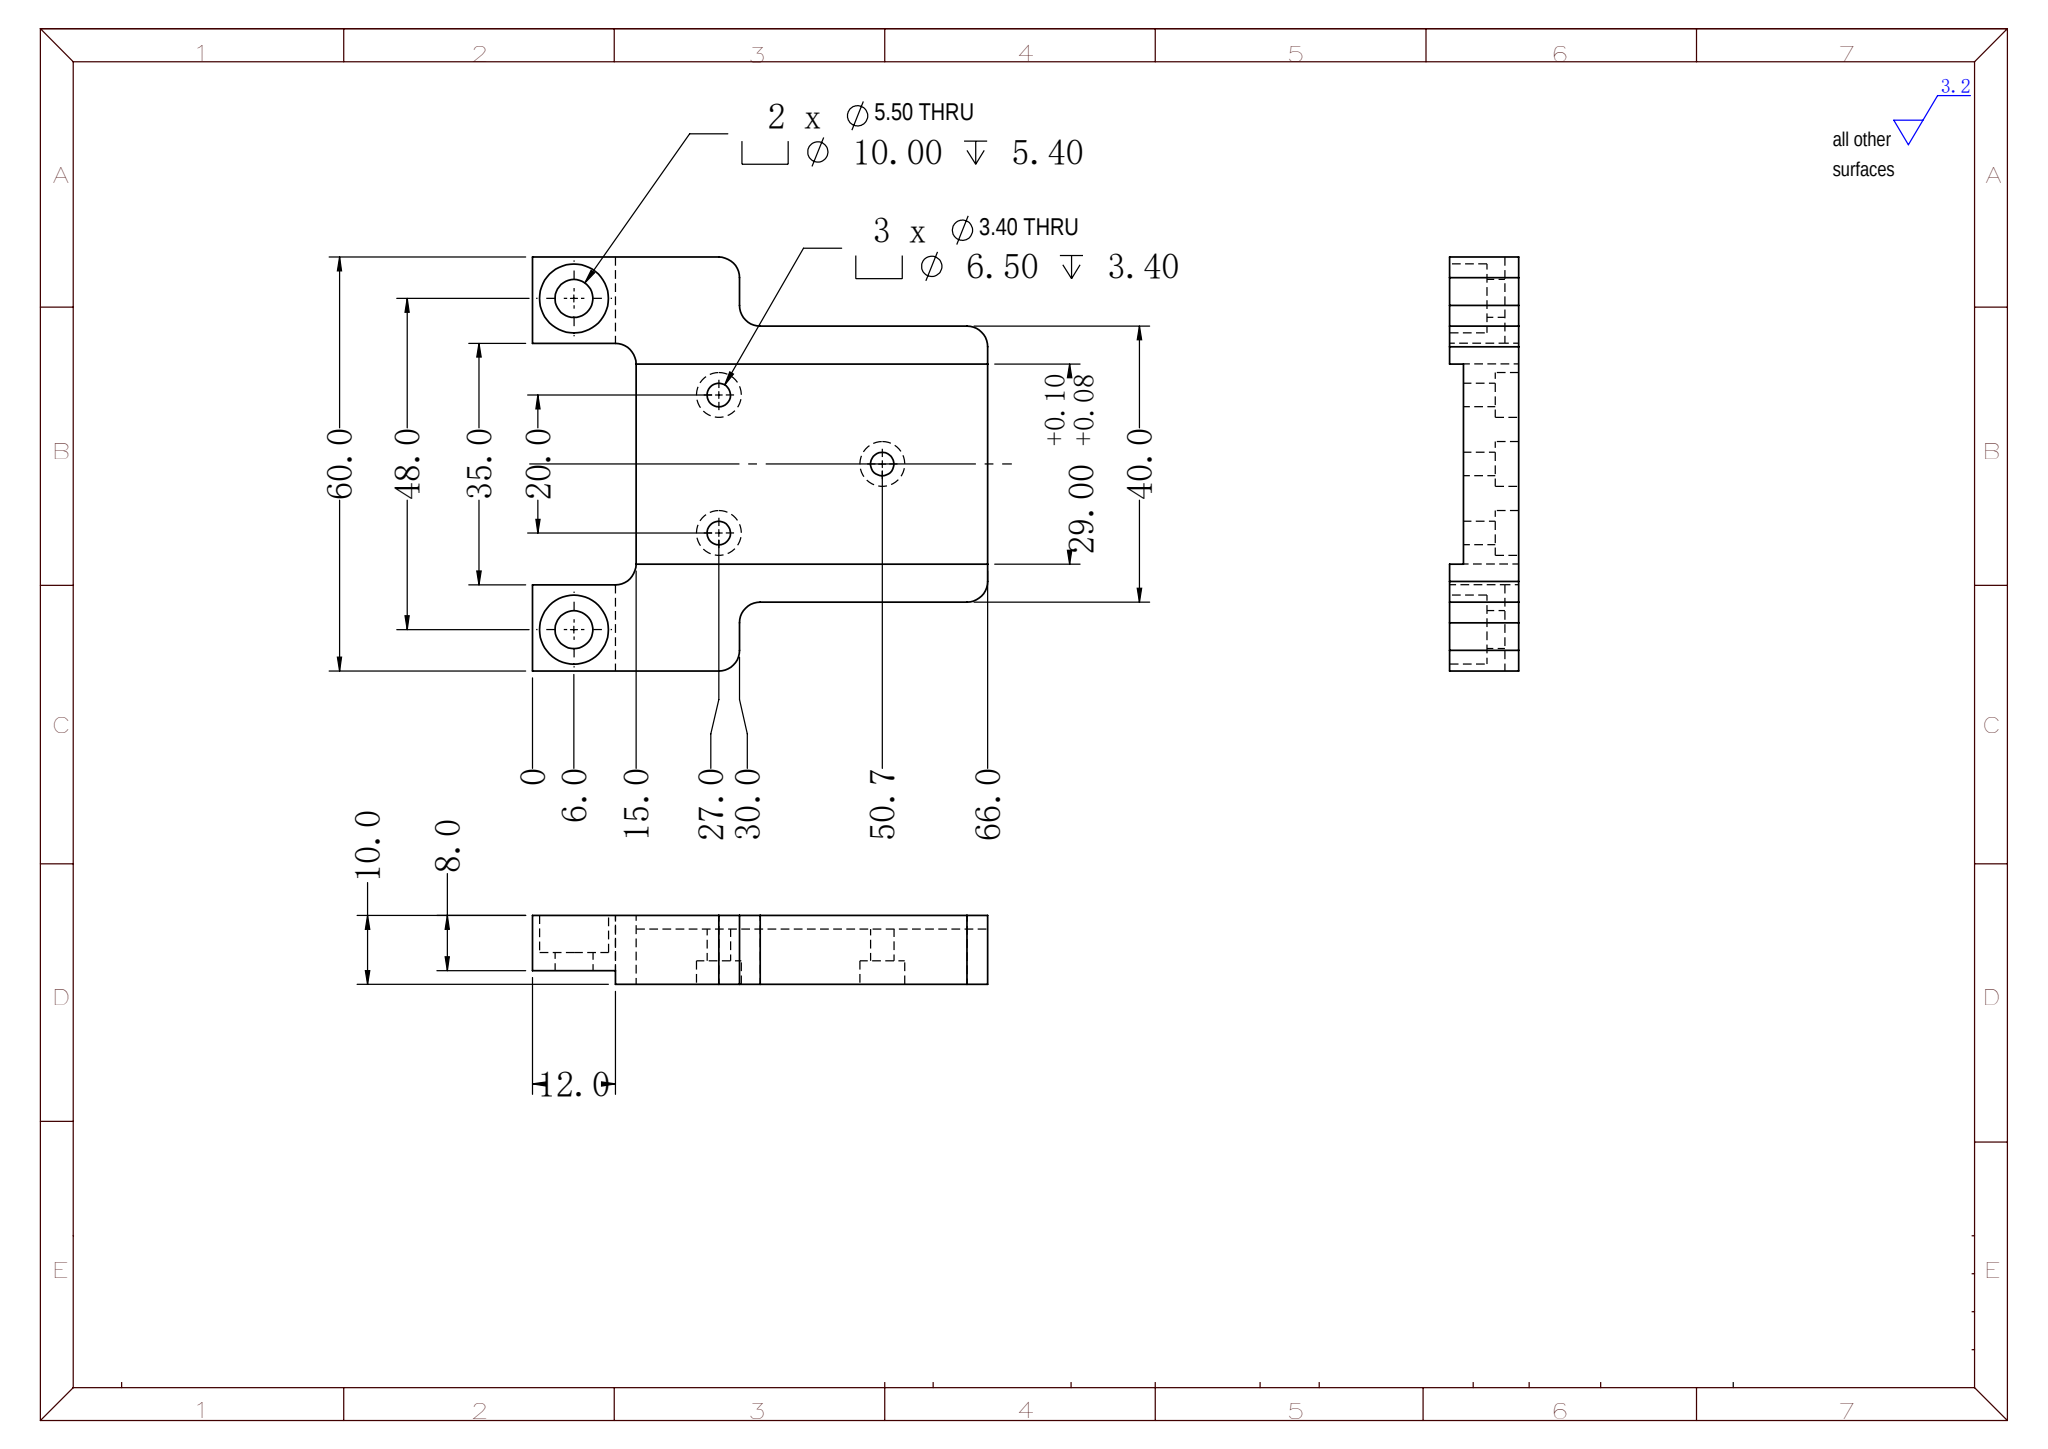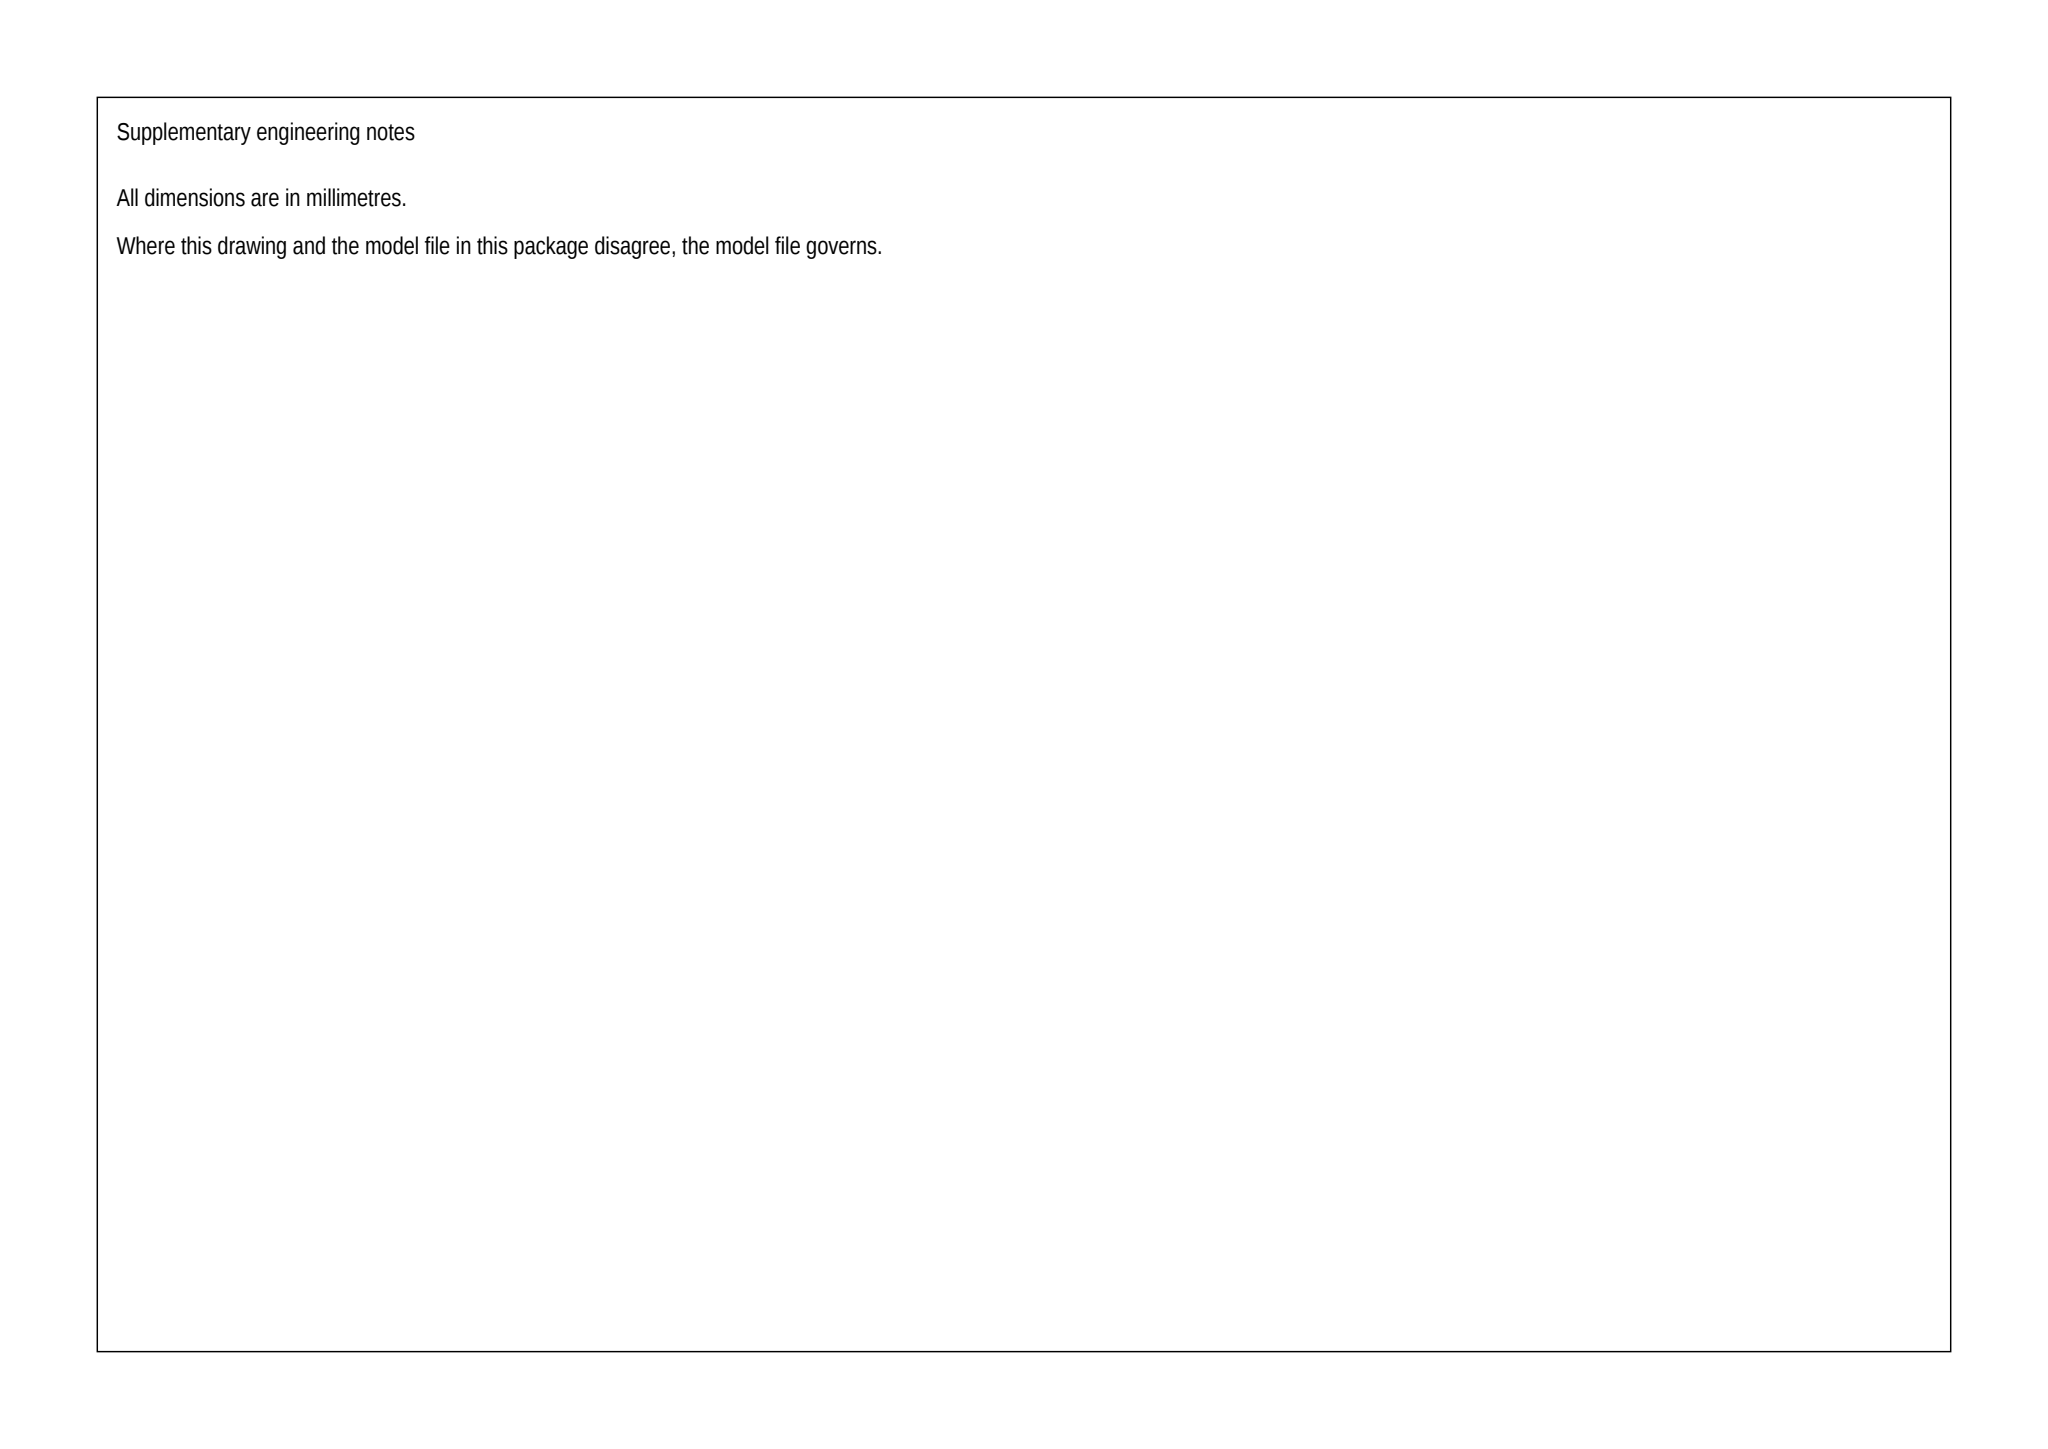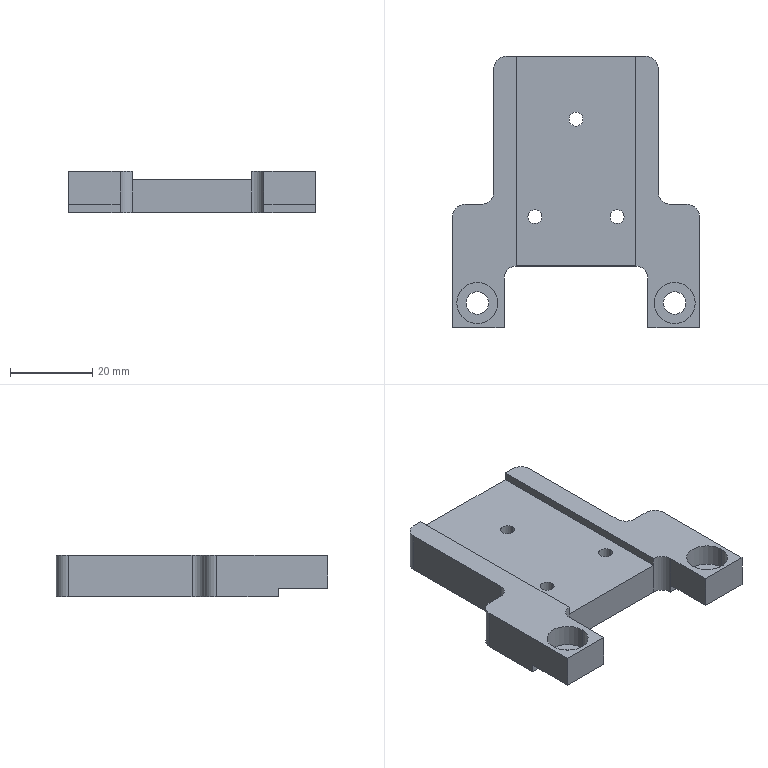Part | SolidWorks | mm | 1 solid | 55 faces | box 60 x 66 x 10 mm | volume 22156 mm3 | cylinder 28 | plane 27 | commonest cylinder face diameters 6 x8 6.5 x6 3.4 x6 10 x4 5.5 x4
build123d program:
from build123d import *

# Parameters (mm, degrees)
BOSS_EXTRUDE1_DEPTH                             = 5
SKETCH30_W                                      = 29
SKETCH30_H                                      = 51
CUT_EXTRUDE15_DEPTH                             = 2
CUT_EXTRUDE16_DEPTH                             = 73.67
CUT_EXTRUDE16_DEPTH_BACK                        = 73.67
SKETCH31_W                                      = 2
SKETCH31_H                                      = 12
M3_HEX_SOCKET_HEAD_CAP_SCREW_CBORE1_D           = 3.4
M3_HEX_SOCKET_HEAD_CAP_SCREW_CBORE1_CBORE_D     = 6.5
M3_HEX_SOCKET_HEAD_CAP_SCREW_CBORE1_CBORE_DEPTH = 3.4
M5_HEX_SOCKET_HEAD_CAP_SCREW_CBORE1_D           = 5.5
M5_HEX_SOCKET_HEAD_CAP_SCREW_CBORE1_CBORE_D     = 10
M5_HEX_SOCKET_HEAD_CAP_SCREW_CBORE1_CBORE_DEPTH = 5.4
FILLET1_R                                       = 3


with BuildPart() as part:
    # Sketch29 → Boss-Extrude1 (new, symmetric)
    with BuildSketch(Plane.XY):
        Polygon((30, 0), (17.5, 0), (17.5, 15), (-17.5, 15), (-17.5, 0), (-30, 0), (-30, 30), (-20, 30), (-20, 66), (20, 66), (20, 30), (30, 30), align=None)
    extrude(amount=BOSS_EXTRUDE1_DEPTH, both=True)

    # Sketch30 → Cut-Extrude15 (cut)
    with BuildSketch(Plane.XY.offset(5)):
        with Locations((0, 40.5)):
            Rectangle(SKETCH30_W, SKETCH30_H)
    extrude(amount=-CUT_EXTRUDE15_DEPTH, mode=Mode.SUBTRACT)

    # Sketch31 → Cut-Extrude16 (cut, two sides: drawn at the far end of the back side and taken through both)
    with BuildSketch(Plane(origin=(0, 0, 0), x_dir=(0, 0, -1), z_dir=(1, 0, 0)).offset(-CUT_EXTRUDE16_DEPTH_BACK)):
        with Locations((4, 6)):
            Rectangle(SKETCH31_W, SKETCH31_H)
    extrude(amount=CUT_EXTRUDE16_DEPTH + CUT_EXTRUDE16_DEPTH_BACK, mode=Mode.SUBTRACT)

    # M3 Hex Socket Head Cap Screw CBORE1 (through all)
    with Locations(Plane(origin=(0, 0, -5), x_dir=(-1, 0, 0), z_dir=(0, 0, -1))):
        with Locations((0, 50.7), (10, 27), (-10, 27)):
            CounterBoreHole(M3_HEX_SOCKET_HEAD_CAP_SCREW_CBORE1_D / 2, M3_HEX_SOCKET_HEAD_CAP_SCREW_CBORE1_CBORE_D / 2, M3_HEX_SOCKET_HEAD_CAP_SCREW_CBORE1_CBORE_DEPTH)

    # M5 Hex Socket Head Cap Screw CBORE1 (through all)
    with Locations(Plane.XY.offset(5)):
        with Locations((24, 6), (-24, 6)):
            CounterBoreHole(M5_HEX_SOCKET_HEAD_CAP_SCREW_CBORE1_D / 2, M5_HEX_SOCKET_HEAD_CAP_SCREW_CBORE1_CBORE_D / 2, M5_HEX_SOCKET_HEAD_CAP_SCREW_CBORE1_CBORE_DEPTH)

    # Fillet1
    fillet1_edges = [part.edges().sort_by_distance(p)[0] for p in [
        (30, 30, 0),
        (20, 66, 0),
        (-20, 66, 0),
        (-30, 30, 0),
        (-20, 30, 0),
        (20, 30, 0),
        (-17.5, 15, 0),
        (17.5, 15, 0),
    ]]
    fillet(fillet1_edges, radius=FILLET1_R)


solid = part.part